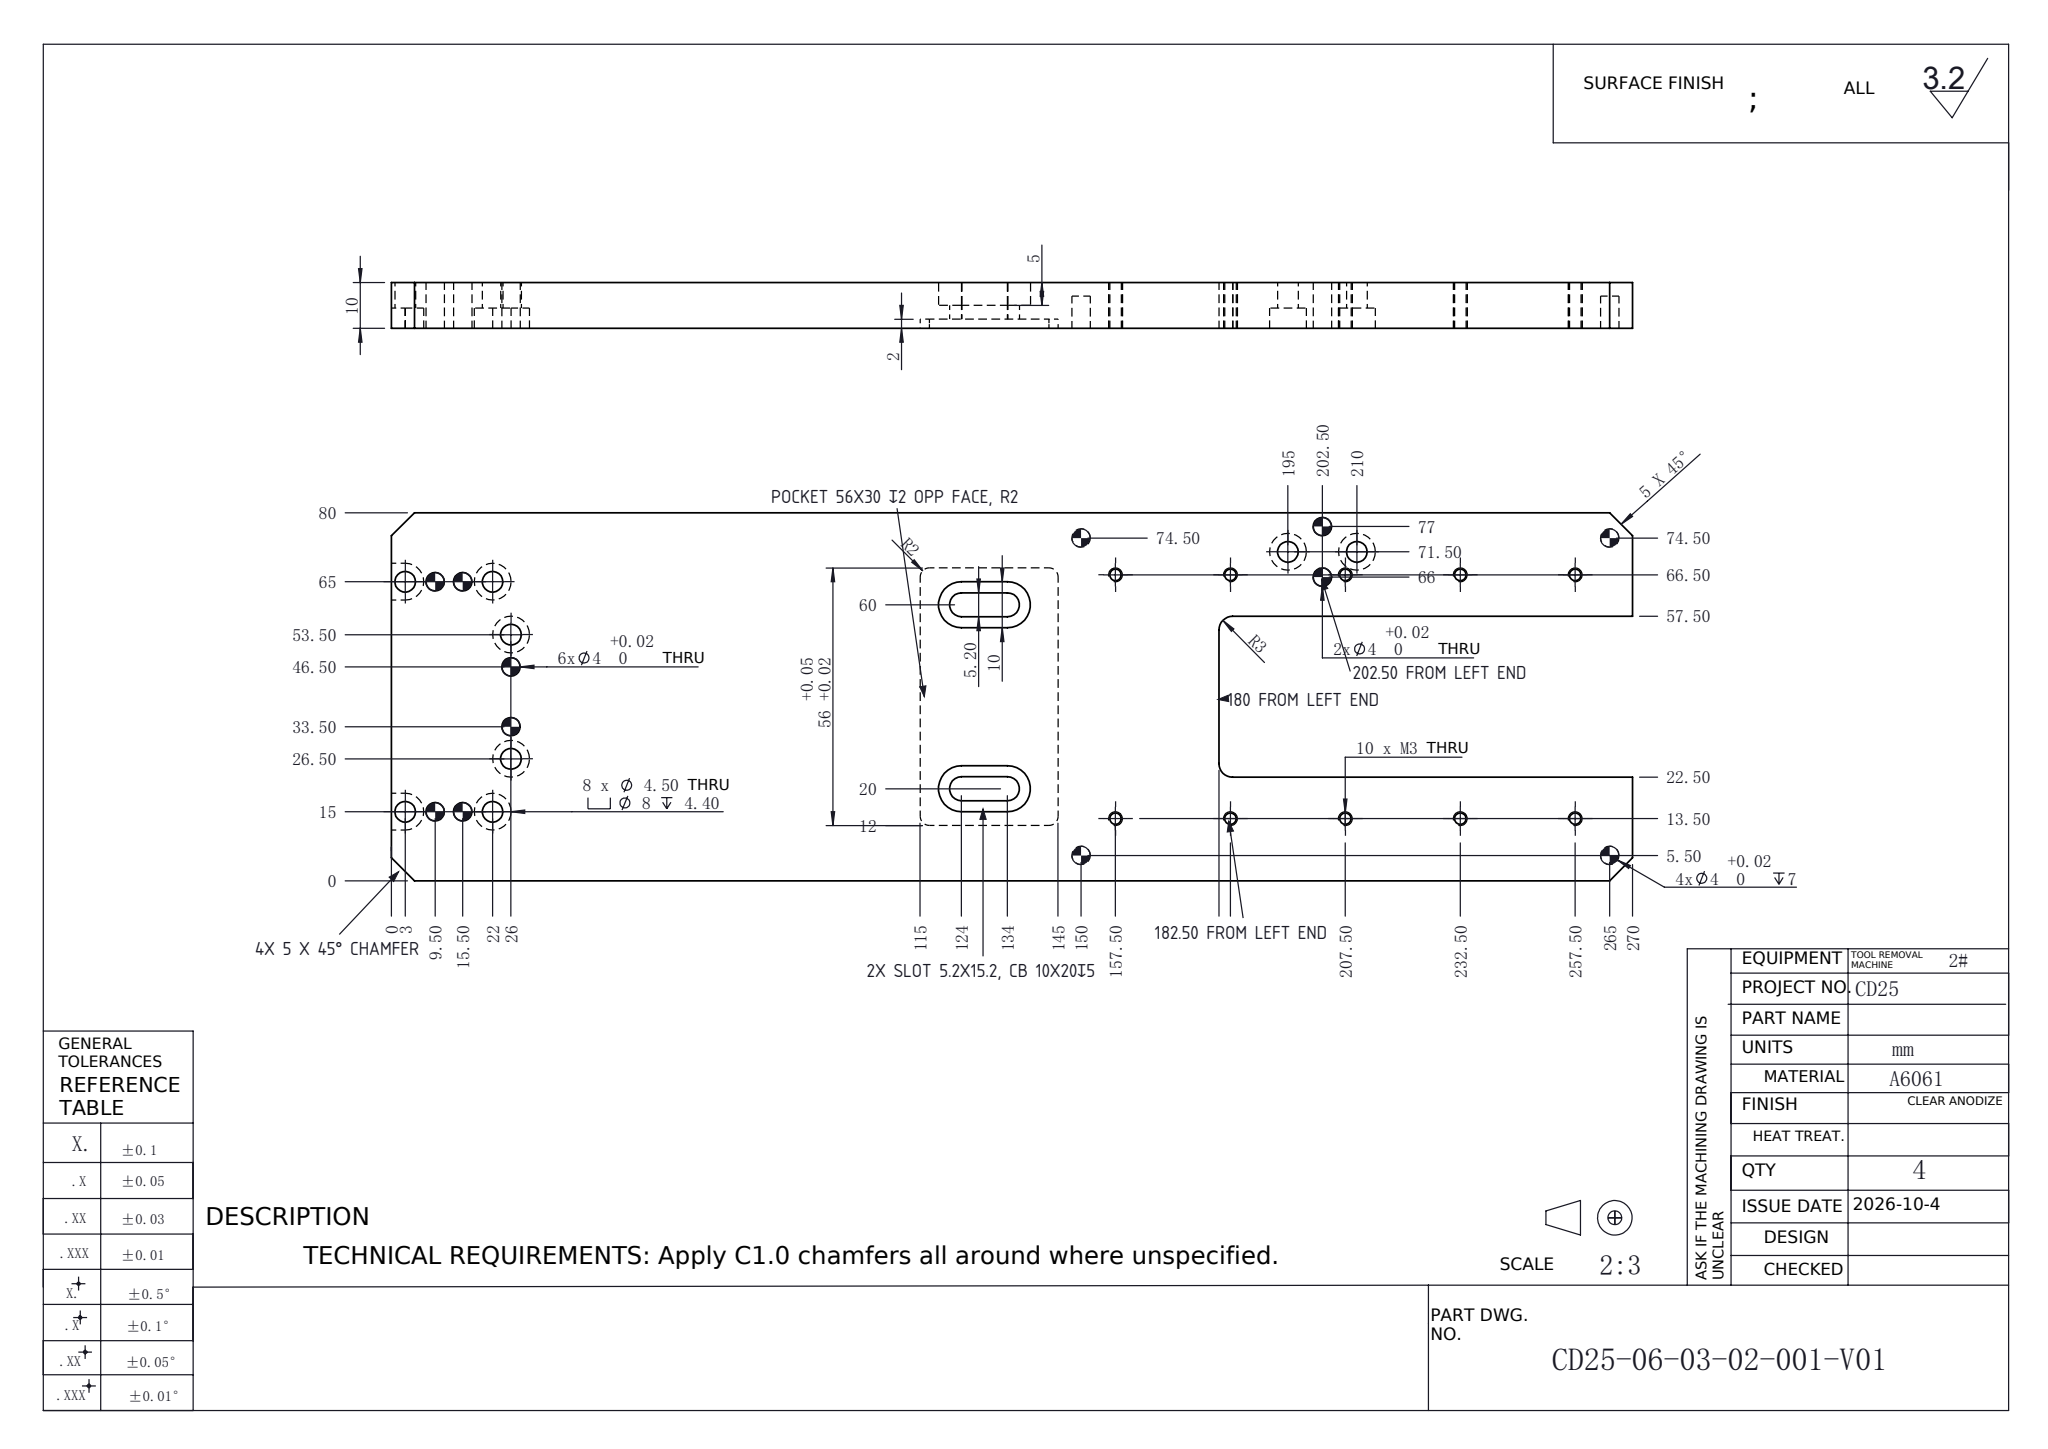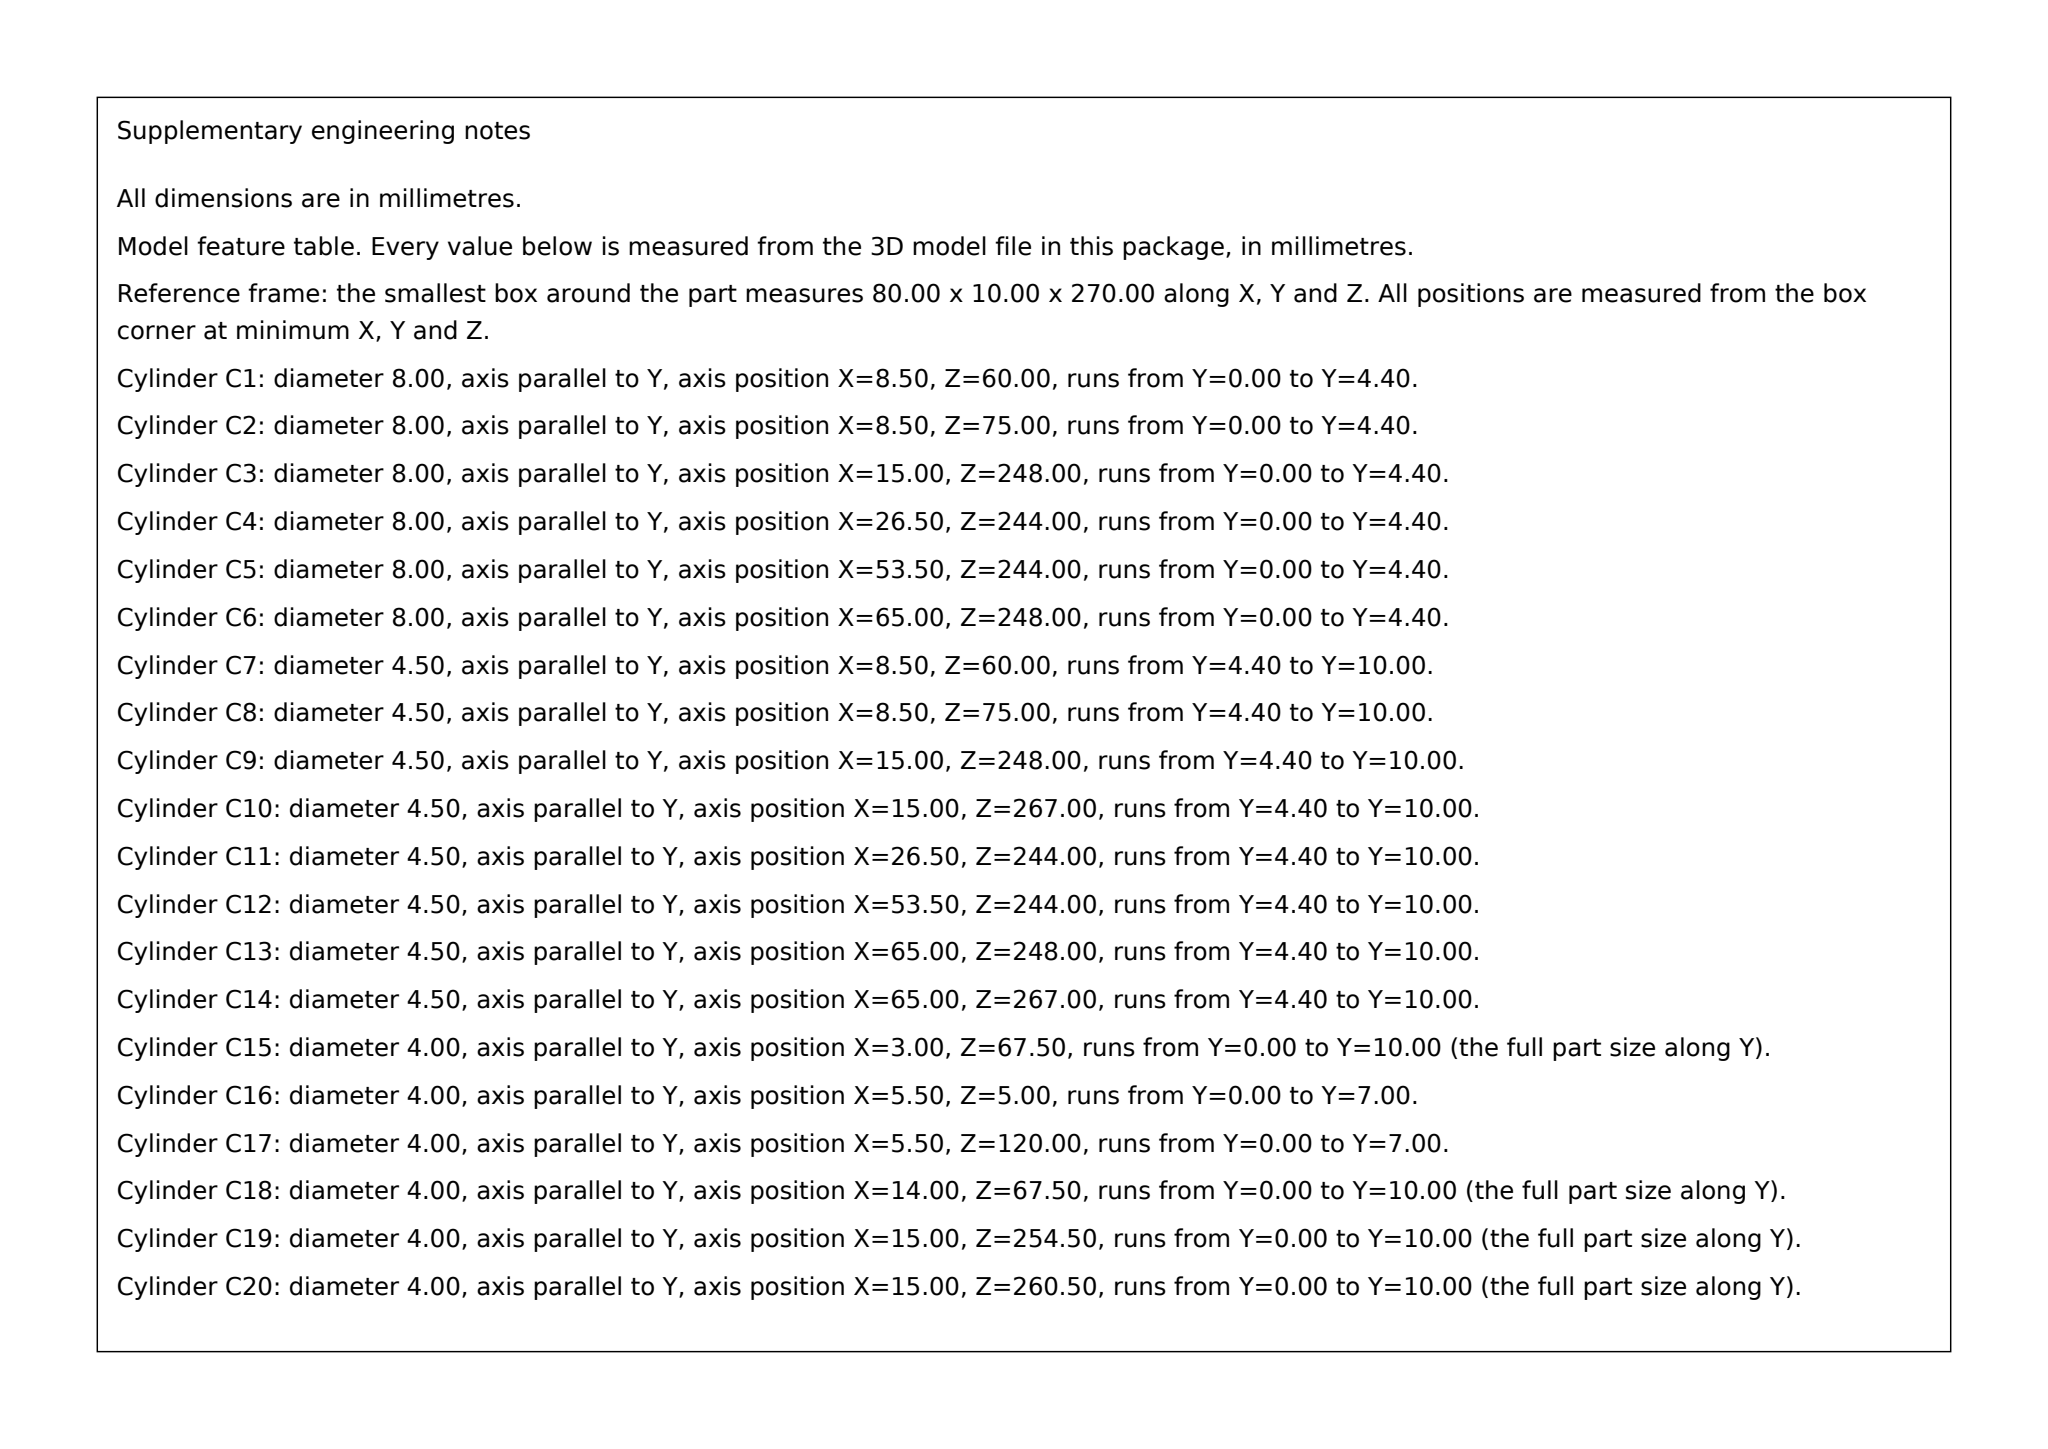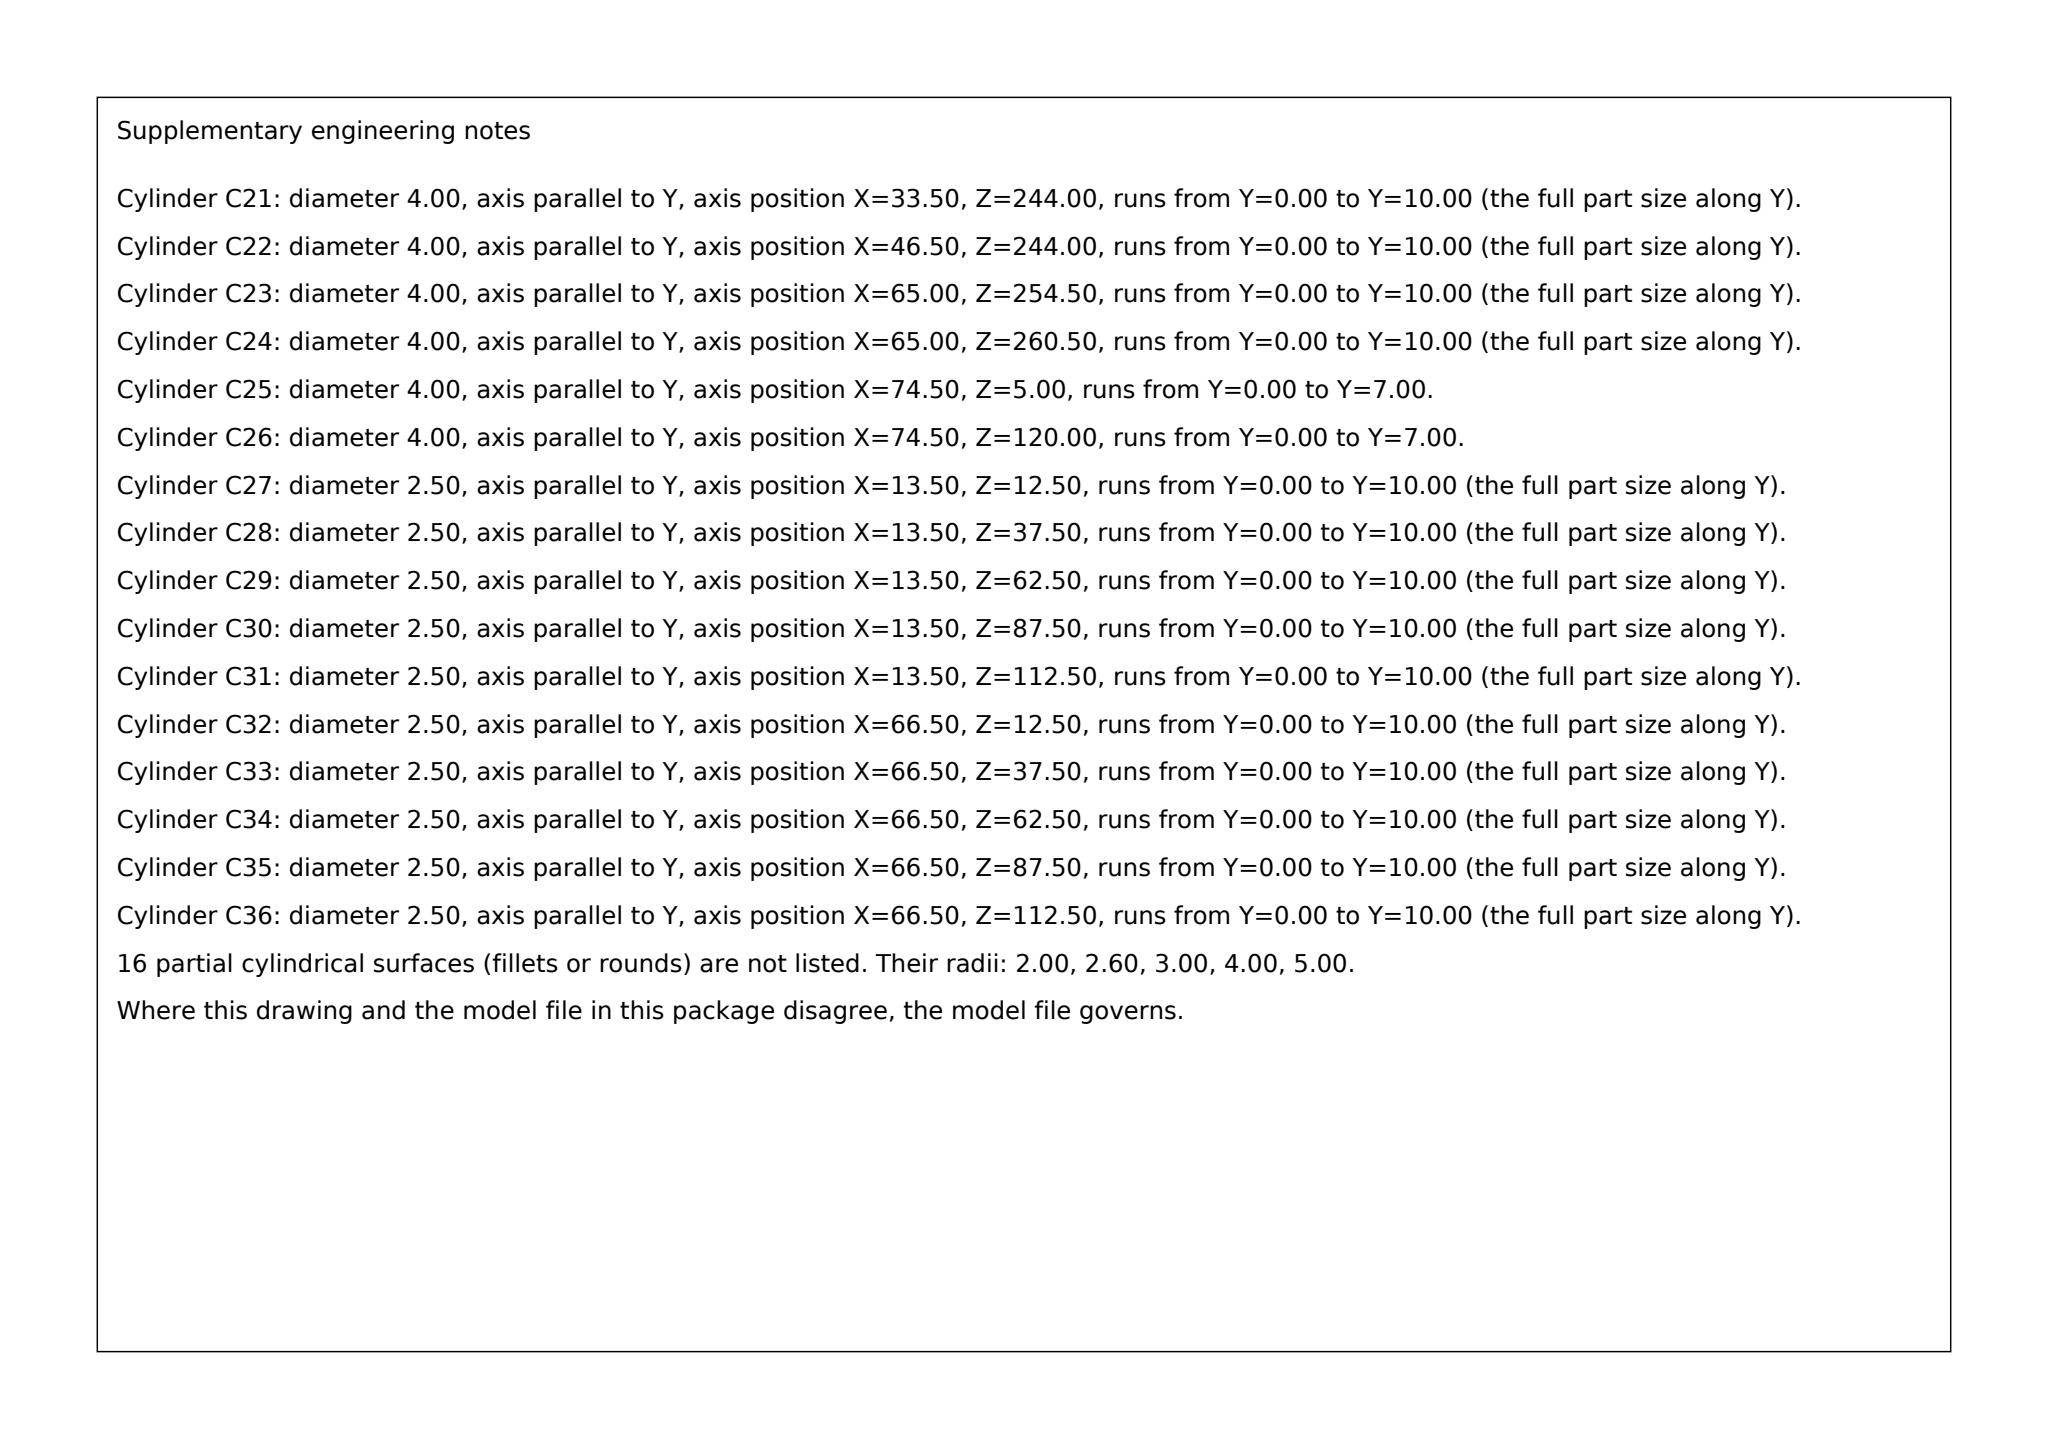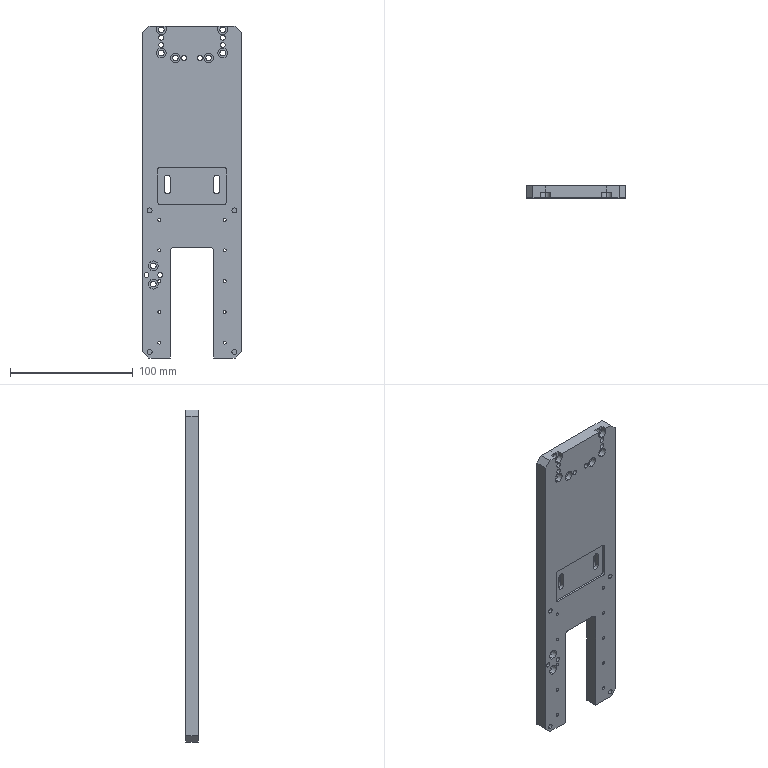Part | SolidWorks | mm | material A6061 | 1 solid | 139 faces | box 80 x 10 x 270 mm | volume 174141 mm3 | cylinder 94 | plane 45 | commonest cylinder face diameters 4 x28 2.5 x20 4.5 x16 8 x16 10 x6 5.2 x6 6 x2
Drawing notes:
POCKET 56 W X 30 LG (Z125-155) DP 2 FROM OPP FACE, R2 CORNERS | from the solid: x planes 12.0 & 68.0 (56 W), z planes 125.0 & 155.0 (30 LG), y plane 2.0; Ø4 corner cyls at x14/66, z127/153, len 2.0
2X SLOT 5.20 W X 15.20 LG THRU, CBORE 10 W X 20 LG DP 5 | from the solid: Ø5.2 cyls len 3.0 and Ø10 cyls len 5.0 at x=20 & 60, z=136 & 146 (10 CRS)
4X 5 X 45° CHAMFER AT PLATE CORNERS (TYP ALL 4) | from the solid: Bbox 270 x 80 plate; four 45° corner cuts, each 5 x 5 flats off x=0/80 and z=0/270 edges (non-axis faces, matching the called-out top-right 5 X 45°)
M3 THRU hole column (rows 13.50 and 66.50 from bottom edge) located 182.50 from left end of plate; part of the 10X M3 THRU pattern at 157.50 / 182.50 / 207.50 / 232.50 / 257.50. | from the solid: cylinders[2.5,"y",[13.5,null,87.5],10.0] and [2.5,"y",[66.5,null,87.5],10.0] -> 270-87.5 = 182.50 from left end
Outline step face (vertical profile edge) located 180 from left end of plate. | from the solid: axis_planes["z",90.0] -> 270-90 = 180 from left end
2X Ø4 +0.02/0 THRU, on column 202.50 from left end of plate; holes at 66.00 and 77.00 from bottom edge. | from the solid: cylinders dia 4.0 axis y, length 10.0 (full 10 mm plate thickness) at [3.0,null,67.5] and [14.0,null,67.5]; bbox 80 x 10 x 270 -> drawing position 270-67.5=202.50 from left end, 80-3=77.00 and 80-14=66.00 from bottom edge